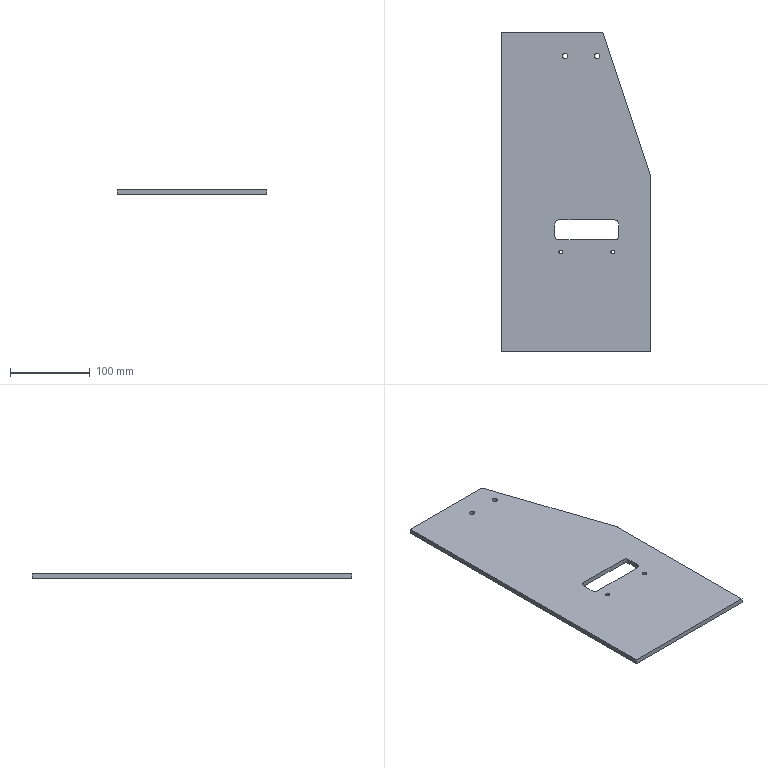Component | SolidWorks | JHK-B1003RightRearBaffle-1 | 1 solid | 25 faces | box 187 x 400 x 6 mm | volume 403848 mm3 | cylinder 14 | plane 11 | commonest cylinder face diameters 5 x4 6.8 x4 10 x4 8 x2 | material Q235A
build123d program:
from build123d import *

# Parameters (mm, degrees)
BOSS_EXTRUDE1_DEPTH = 3
M8_TAPPED_HOLE1_D   = 6.8
FILLET1_R           = 4
CUT_EXTRUDE3_DEPTH  = 221.858
M6_TAPPED_HOLE1_D   = 5


with BuildPart() as part:
    # Sketch1 → Boss-Extrude1 (new, symmetric)
    with BuildSketch(Plane.XY):
        Polygon((93.5, 200), (-33.5, 200), (-93.5, 20), (-93.5, -200), (93.5, -200), align=None)
    extrude(amount=BOSS_EXTRUDE1_DEPTH, both=True)

    # M8 Tapped Hole1 (through all)
    with Locations(Plane.XY.offset(3)):
        with Locations((13.5, 170), (-26.5, 170)):
            Hole(M8_TAPPED_HOLE1_D / 2)

    # Fillet1
    fillet1_edges = [part.edges().sort_by_distance(p)[0] for p in [
        (-93.5, 20, 0),
        (-33.5, 200, 0),
    ]]
    fillet(fillet1_edges, radius=FILLET1_R)

    # Sketch6 → Cut-Extrude3 (cut, through all)
    with BuildSketch(Plane.XY.offset(3)):
        with BuildLine():
            Line((-48.5, -60), (21.5, -60))
            ThreePointArc((21.5, -60), (25.036, -58.536), (26.5, -55))
            Line((26.5, -55), (26.5, -40))
            ThreePointArc((26.5, -40), (25.036, -36.464), (21.5, -35))
            Line((21.5, -35), (-48.5, -35))
            ThreePointArc((-48.5, -35), (-52.036, -36.464), (-53.5, -40))
            Line((-53.5, -40), (-53.5, -55))
            ThreePointArc((-53.5, -55), (-52.036, -58.536), (-48.5, -60))
        make_face()
    extrude(amount=-CUT_EXTRUDE3_DEPTH, mode=Mode.SUBTRACT)

    # M6 Tapped Hole1 (through all)
    with Locations(Plane.XY.offset(3)):
        with Locations((-46, -75), (19, -75)):
            Hole(M6_TAPPED_HOLE1_D / 2)


solid = part.part

# Placed as in the assembly
solid = solid.moved(Location((226.5, 0, -142), (-180, 0, 180)))
STEP:
#1=COLOUR_RGB('',0.7922,0.8196,0.9333);
#2=FILL_AREA_STYLE_COLOUR('',#1);
#3=FILL_AREA_STYLE('',(#2));
#4=SURFACE_STYLE_FILL_AREA(#3);
#5=SURFACE_SIDE_STYLE('',(#4));
#6=SURFACE_STYLE_USAGE(.BOTH.,#5);
#7=PRESENTATION_STYLE_ASSIGNMENT((#6));
#8=CARTESIAN_POINT('',(10.827,-2.953,-5.472));
#9=VERTEX_POINT('',#8);
#10=CARTESIAN_POINT('',(10.63,-2.953,-5.472));
#11=VERTEX_POINT('',#10);
#12=CARTESIAN_POINT('',(10.728,-2.953,-5.472));
#13=DIRECTION('',(0.,0.,-1.));
#14=DIRECTION('',(-1.,0.,0.));
#15=AXIS2_PLACEMENT_3D('',#12,#13,#14);
#16=CIRCLE('',#15,0.09843);
#17=EDGE_CURVE('',#9,#11,#16,.T.);
#18=ORIENTED_EDGE('',*,*,#17,.F.);
#19=CARTESIAN_POINT('',(10.827,-2.953,-5.709));
#20=VERTEX_POINT('',#19);
#21=CARTESIAN_POINT('',(10.827,-2.953,-5.709));
#22=DIRECTION('',(0.,0.,-1.));
#23=VECTOR('',#22,39.37);
#24=LINE('',#21,#23);
#25=EDGE_CURVE('',#9,#20,#24,.T.);
#26=ORIENTED_EDGE('',*,*,#25,.T.);
#27=CARTESIAN_POINT('',(10.63,-2.953,-5.709));
#28=VERTEX_POINT('',#27);
#29=CARTESIAN_POINT('',(10.728,-2.953,-5.709));
#30=DIRECTION('',(0.,0.,-1.));
#31=DIRECTION('',(-1.,0.,0.));
#32=AXIS2_PLACEMENT_3D('',#29,#30,#31);
#33=CIRCLE('',#32,0.09843);
#34=EDGE_CURVE('',#20,#28,#33,.T.);
#35=ORIENTED_EDGE('',*,*,#34,.T.);
#36=CARTESIAN_POINT('',(10.63,-2.953,-5.709));
#37=DIRECTION('',(0.,0.,-1.));
#38=VECTOR('',#37,39.37);
#39=LINE('',#36,#38);
#40=EDGE_CURVE('',#11,#28,#39,.T.);
#41=ORIENTED_EDGE('',*,*,#40,.F.);
#42=EDGE_LOOP('',(#18,#26,#35,#41));
#43=FACE_OUTER_BOUND('',#42,.T.);
#44=CARTESIAN_POINT('',(10.728,-2.953,-5.709));
#45=DIRECTION('',(0.,0.,-1.));
#46=DIRECTION('',(-1.,0.,0.));
#47=AXIS2_PLACEMENT_3D('',#44,#45,#46);
#48=CYLINDRICAL_SURFACE('',#47,0.09843);
#49=ADVANCED_FACE('',(#43),#48,.F.);
#50=CARTESIAN_POINT('',(8.268,-2.953,-5.472));
#51=VERTEX_POINT('',#50);
#52=CARTESIAN_POINT('',(8.071,-2.953,-5.472));
#53=VERTEX_POINT('',#52);
#54=CARTESIAN_POINT('',(8.169,-2.953,-5.472));
#55=DIRECTION('',(0.,0.,-1.));
#56=DIRECTION('',(-1.,0.,0.));
#57=AXIS2_PLACEMENT_3D('',#54,#55,#56);
#58=CIRCLE('',#57,0.09843);
#59=EDGE_CURVE('',#51,#53,#58,.T.);
#60=ORIENTED_EDGE('',*,*,#59,.F.);
#61=CARTESIAN_POINT('',(8.268,-2.953,-5.709));
#62=VERTEX_POINT('',#61);
#63=CARTESIAN_POINT('',(8.268,-2.953,-5.709));
#64=DIRECTION('',(0.,0.,-1.));
#65=VECTOR('',#64,39.37);
#66=LINE('',#63,#65);
#67=EDGE_CURVE('',#51,#62,#66,.T.);
#68=ORIENTED_EDGE('',*,*,#67,.T.);
#69=CARTESIAN_POINT('',(8.071,-2.953,-5.709));
#70=VERTEX_POINT('',#69);
#71=CARTESIAN_POINT('',(8.169,-2.953,-5.709));
#72=DIRECTION('',(0.,0.,-1.));
#73=DIRECTION('',(-1.,0.,0.));
#74=AXIS2_PLACEMENT_3D('',#71,#72,#73);
#75=CIRCLE('',#74,0.09843);
#76=EDGE_CURVE('',#62,#70,#75,.T.);
#77=ORIENTED_EDGE('',*,*,#76,.T.);
#78=CARTESIAN_POINT('',(8.071,-2.953,-5.709));
#79=DIRECTION('',(0.,0.,-1.));
#80=VECTOR('',#79,39.37);
#81=LINE('',#78,#80);
#82=EDGE_CURVE('',#53,#70,#81,.T.);
#83=ORIENTED_EDGE('',*,*,#82,.F.);
#84=EDGE_LOOP('',(#60,#68,#77,#83));
#85=FACE_OUTER_BOUND('',#84,.T.);
#86=CARTESIAN_POINT('',(8.169,-2.953,-5.709));
#87=DIRECTION('',(0.,0.,-1.));
#88=DIRECTION('',(-1.,0.,0.));
#89=AXIS2_PLACEMENT_3D('',#86,#87,#88);
#90=CYLINDRICAL_SURFACE('',#89,0.09843);
#91=ADVANCED_FACE('',(#85),#90,.F.);
#92=CARTESIAN_POINT('',(8.52,6.693,-5.472));
#93=VERTEX_POINT('',#92);
#94=CARTESIAN_POINT('',(8.252,6.693,-5.472));
#95=VERTEX_POINT('',#94);
#96=CARTESIAN_POINT('',(8.386,6.693,-5.472));
#97=DIRECTION('',(0.,0.,-1.));
#98=DIRECTION('',(-1.,0.,0.));
#99=AXIS2_PLACEMENT_3D('',#96,#97,#98);
#100=CIRCLE('',#99,0.1339);
#101=EDGE_CURVE('',#93,#95,#100,.T.);
#102=ORIENTED_EDGE('',*,*,#101,.F.);
#103=CARTESIAN_POINT('',(8.52,6.693,-5.709));
#104=VERTEX_POINT('',#103);
#105=CARTESIAN_POINT('',(8.52,6.693,-5.709));
#106=DIRECTION('',(0.,0.,-1.));
#107=VECTOR('',#106,39.37);
#108=LINE('',#105,#107);
#109=EDGE_CURVE('',#93,#104,#108,.T.);
#110=ORIENTED_EDGE('',*,*,#109,.T.);
#111=CARTESIAN_POINT('',(8.252,6.693,-5.709));
#112=VERTEX_POINT('',#111);
#113=CARTESIAN_POINT('',(8.386,6.693,-5.709));
#114=DIRECTION('',(0.,0.,-1.));
#115=DIRECTION('',(-1.,0.,0.));
#116=AXIS2_PLACEMENT_3D('',#113,#114,#115);
#117=CIRCLE('',#116,0.1339);
#118=EDGE_CURVE('',#104,#112,#117,.T.);
#119=ORIENTED_EDGE('',*,*,#118,.T.);
#120=CARTESIAN_POINT('',(8.252,6.693,-5.709));
#121=DIRECTION('',(0.,0.,-1.));
#122=VECTOR('',#121,39.37);
#123=LINE('',#120,#122);
#124=EDGE_CURVE('',#95,#112,#123,.T.);
#125=ORIENTED_EDGE('',*,*,#124,.F.);
#126=EDGE_LOOP('',(#102,#110,#119,#125));
#127=FACE_OUTER_BOUND('',#126,.T.);
#128=CARTESIAN_POINT('',(8.386,6.693,-5.709));
#129=DIRECTION('',(0.,0.,-1.));
#130=DIRECTION('',(-1.,0.,0.));
#131=AXIS2_PLACEMENT_3D('',#128,#129,#130);
#132=CYLINDRICAL_SURFACE('',#131,0.1339);
#133=ADVANCED_FACE('',(#127),#132,.F.);
#134=CARTESIAN_POINT('',(10.094,6.693,-5.472));
#135=VERTEX_POINT('',#134);
#136=CARTESIAN_POINT('',(9.827,6.693,-5.472));
#137=VERTEX_POINT('',#136);
#138=CARTESIAN_POINT('',(9.961,6.693,-5.472));
#139=DIRECTION('',(0.,0.,-1.));
#140=DIRECTION('',(-1.,0.,0.));
#141=AXIS2_PLACEMENT_3D('',#138,#139,#140);
#142=CIRCLE('',#141,0.1339);
#143=EDGE_CURVE('',#135,#137,#142,.T.);
#144=ORIENTED_EDGE('',*,*,#143,.F.);
#145=CARTESIAN_POINT('',(10.094,6.693,-5.709));
#146=VERTEX_POINT('',#145);
#147=CARTESIAN_POINT('',(10.094,6.693,-5.709));
#148=DIRECTION('',(0.,0.,-1.));
#149=VECTOR('',#148,39.37);
#150=LINE('',#147,#149);
#151=EDGE_CURVE('',#135,#146,#150,.T.);
#152=ORIENTED_EDGE('',*,*,#151,.T.);
#153=CARTESIAN_POINT('',(9.827,6.693,-5.709));
#154=VERTEX_POINT('',#153);
#155=CARTESIAN_POINT('',(9.961,6.693,-5.709));
#156=DIRECTION('',(0.,0.,-1.));
#157=DIRECTION('',(-1.,0.,0.));
#158=AXIS2_PLACEMENT_3D('',#155,#156,#157);
#159=CIRCLE('',#158,0.1339);
#160=EDGE_CURVE('',#146,#154,#159,.T.);
#161=ORIENTED_EDGE('',*,*,#160,.T.);
#162=CARTESIAN_POINT('',(9.827,6.693,-5.709));
#163=DIRECTION('',(0.,0.,-1.));
#164=VECTOR('',#163,39.37);
#165=LINE('',#162,#164);
#166=EDGE_CURVE('',#137,#154,#165,.T.);
#167=ORIENTED_EDGE('',*,*,#166,.F.);
#168=EDGE_LOOP('',(#144,#152,#161,#167));
#169=FACE_OUTER_BOUND('',#168,.T.);
#170=CARTESIAN_POINT('',(9.961,6.693,-5.709));
#171=DIRECTION('',(0.,0.,-1.));
#172=DIRECTION('',(-1.,0.,0.));
#173=AXIS2_PLACEMENT_3D('',#170,#171,#172);
#174=CYLINDRICAL_SURFACE('',#173,0.1339);
#175=ADVANCED_FACE('',(#169),#174,.F.);
#176=CARTESIAN_POINT('',(12.598,0.7618,-5.709));
#177=VERTEX_POINT('',#176);
#178=CARTESIAN_POINT('',(12.598,-7.874,-5.709));
#179=VERTEX_POINT('',#178);
#180=CARTESIAN_POINT('',(12.598,-7.874,-5.709));
#181=DIRECTION('',(0.,-1.,0.));
#182=VECTOR('',#181,39.37);
#183=LINE('',#180,#182);
#184=EDGE_CURVE('',#177,#179,#183,.T.);
#185=ORIENTED_EDGE('',*,*,#184,.F.);
#186=CARTESIAN_POINT('',(12.598,0.7618,-5.472));
#187=VERTEX_POINT('',#186);
#188=CARTESIAN_POINT('',(12.598,0.7618,-5.709));
#189=DIRECTION('',(-0.,-0.,1.));
#190=VECTOR('',#189,39.37);
#191=LINE('',#188,#190);
#192=EDGE_CURVE('',#177,#187,#191,.T.);
#193=ORIENTED_EDGE('',*,*,#192,.T.);
#194=CARTESIAN_POINT('',(12.598,-7.874,-5.472));
#195=VERTEX_POINT('',#194);
#196=CARTESIAN_POINT('',(12.598,-7.874,-5.472));
#197=DIRECTION('',(0.,-1.,0.));
#198=VECTOR('',#197,39.37);
#199=LINE('',#196,#198);
#200=EDGE_CURVE('',#187,#195,#199,.T.);
#201=ORIENTED_EDGE('',*,*,#200,.T.);
#202=CARTESIAN_POINT('',(12.598,-7.874,-5.709));
#203=DIRECTION('',(-0.,-0.,1.));
#204=VECTOR('',#203,39.37);
#205=LINE('',#202,#204);
#206=EDGE_CURVE('',#179,#195,#205,.T.);
#207=ORIENTED_EDGE('',*,*,#206,.F.);
#208=EDGE_LOOP('',(#185,#193,#201,#207));
#209=FACE_OUTER_BOUND('',#208,.T.);
#210=CARTESIAN_POINT('',(12.598,-7.874,-5.709));
#211=DIRECTION('',(-1.,-0.,-0.));
#212=DIRECTION('',(-0.,-0.,1.));
#213=AXIS2_PLACEMENT_3D('',#210,#211,#212);
#214=PLANE('',#213);
#215=ADVANCED_FACE('',(#209),#214,.F.);
#216=CARTESIAN_POINT('',(5.236,-7.874,-5.472));
#217=VERTEX_POINT('',#216);
#218=CARTESIAN_POINT('',(12.598,-7.874,-5.472));
#219=DIRECTION('',(-1.,-0.,0.));
#220=VECTOR('',#219,39.37);
#221=LINE('',#218,#220);
#222=EDGE_CURVE('',#195,#217,#221,.T.);
#223=ORIENTED_EDGE('',*,*,#222,.T.);
#224=CARTESIAN_POINT('',(5.236,-7.874,-5.709));
#225=VERTEX_POINT('',#224);
#226=CARTESIAN_POINT('',(5.236,-7.874,-5.709));
#227=DIRECTION('',(-0.,-0.,1.));
#228=VECTOR('',#227,39.37);
#229=LINE('',#226,#228);
#230=EDGE_CURVE('',#225,#217,#229,.T.);
#231=ORIENTED_EDGE('',*,*,#230,.F.);
#232=CARTESIAN_POINT('',(12.598,-7.874,-5.709));
#233=DIRECTION('',(-1.,-0.,0.));
#234=VECTOR('',#233,39.37);
#235=LINE('',#232,#234);
#236=EDGE_CURVE('',#179,#225,#235,.T.);
#237=ORIENTED_EDGE('',*,*,#236,.F.);
#238=ORIENTED_EDGE('',*,*,#206,.T.);
#239=EDGE_LOOP('',(#223,#231,#237,#238));
#240=FACE_OUTER_BOUND('',#239,.T.);
#241=CARTESIAN_POINT('',(12.598,-7.874,-5.709));
#242=DIRECTION('',(-0.,1.,0.));
#243=DIRECTION('',(0.,0.,-1.));
#244=AXIS2_PLACEMENT_3D('',#241,#242,#243);
#245=PLANE('',#244);
#246=ADVANCED_FACE('',(#240),#245,.F.);
#247=CARTESIAN_POINT('',(5.236,7.874,-5.472));
#248=VERTEX_POINT('',#247);
#249=CARTESIAN_POINT('',(5.236,7.874,-5.472));
#250=DIRECTION('',(-0.,1.,-0.));
#251=VECTOR('',#250,39.37);
#252=LINE('',#249,#251);
#253=EDGE_CURVE('',#217,#248,#252,.T.);
#254=ORIENTED_EDGE('',*,*,#253,.T.);
#255=CARTESIAN_POINT('',(5.236,7.874,-5.709));
#256=VERTEX_POINT('',#255);
#257=CARTESIAN_POINT('',(5.236,7.874,-5.709));
#258=DIRECTION('',(-0.,-0.,1.));
#259=VECTOR('',#258,39.37);
#260=LINE('',#257,#259);
#261=EDGE_CURVE('',#256,#248,#260,.T.);
#262=ORIENTED_EDGE('',*,*,#261,.F.);
#263=CARTESIAN_POINT('',(5.236,7.874,-5.709));
#264=DIRECTION('',(-0.,1.,-0.));
#265=VECTOR('',#264,39.37);
#266=LINE('',#263,#265);
#267=EDGE_CURVE('',#225,#256,#266,.T.);
#268=ORIENTED_EDGE('',*,*,#267,.F.);
#269=ORIENTED_EDGE('',*,*,#230,.T.);
#270=EDGE_LOOP('',(#254,#262,#268,#269));
#271=FACE_OUTER_BOUND('',#270,.T.);
#272=CARTESIAN_POINT('',(5.236,7.874,-5.709));
#273=DIRECTION('',(1.,0.,0.));
#274=DIRECTION('',(0.,0.,-1.));
#275=AXIS2_PLACEMENT_3D('',#272,#273,#274);
#276=PLANE('',#275);
#277=ADVANCED_FACE('',(#271),#276,.F.);
#278=CARTESIAN_POINT('',(10.123,7.874,-5.472));
#279=VERTEX_POINT('',#278);
#280=CARTESIAN_POINT('',(5.236,7.874,-5.472));
#281=DIRECTION('',(1.,0.,-0.));
#282=VECTOR('',#281,39.37);
#283=LINE('',#280,#282);
#284=EDGE_CURVE('',#248,#279,#283,.T.);
#285=ORIENTED_EDGE('',*,*,#284,.T.);
#286=CARTESIAN_POINT('',(10.123,7.874,-5.709));
#287=VERTEX_POINT('',#286);
#288=CARTESIAN_POINT('',(10.123,7.874,-5.709));
#289=DIRECTION('',(0.,0.,-1.));
#290=VECTOR('',#289,39.37);
#291=LINE('',#288,#290);
#292=EDGE_CURVE('',#279,#287,#291,.T.);
#293=ORIENTED_EDGE('',*,*,#292,.T.);
#294=CARTESIAN_POINT('',(5.236,7.874,-5.709));
#295=DIRECTION('',(1.,0.,-0.));
#296=VECTOR('',#295,39.37);
#297=LINE('',#294,#296);
#298=EDGE_CURVE('',#256,#287,#297,.T.);
#299=ORIENTED_EDGE('',*,*,#298,.F.);
#300=ORIENTED_EDGE('',*,*,#261,.T.);
#301=EDGE_LOOP('',(#285,#293,#299,#300));
#302=FACE_OUTER_BOUND('',#301,.T.);
#303=CARTESIAN_POINT('',(5.236,7.874,-5.709));
#304=DIRECTION('',(0.,-1.,0.));
#305=DIRECTION('',(-1.,-0.,0.));
#306=AXIS2_PLACEMENT_3D('',#303,#304,#305);
#307=PLANE('',#306);
#308=ADVANCED_FACE('',(#302),#307,.F.);
#309=CARTESIAN_POINT('',(10.272,7.766,-5.472));
#310=VERTEX_POINT('',#309);
#311=CARTESIAN_POINT('',(12.59,0.8116,-5.472));
#312=VERTEX_POINT('',#311);
#313=CARTESIAN_POINT('',(12.598,0.7874,-5.472));
#314=DIRECTION('',(0.3162,-0.9487,0.));
#315=VECTOR('',#314,39.37);
#316=LINE('',#313,#315);
#317=EDGE_CURVE('',#310,#312,#316,.T.);
#318=ORIENTED_EDGE('',*,*,#317,.T.);
#319=CARTESIAN_POINT('',(12.59,0.8116,-5.709));
#320=VERTEX_POINT('',#319);
#321=CARTESIAN_POINT('',(12.59,0.8116,-5.709));
#322=DIRECTION('',(0.,0.,-1.));
#323=VECTOR('',#322,39.37);
#324=LINE('',#321,#323);
#325=EDGE_CURVE('',#312,#320,#324,.T.);
#326=ORIENTED_EDGE('',*,*,#325,.T.);
#327=CARTESIAN_POINT('',(10.272,7.766,-5.709));
#328=VERTEX_POINT('',#327);
#329=CARTESIAN_POINT('',(12.598,0.7874,-5.709));
#330=DIRECTION('',(0.3162,-0.9487,0.));
#331=VECTOR('',#330,39.37);
#332=LINE('',#329,#331);
#333=EDGE_CURVE('',#328,#320,#332,.T.);
#334=ORIENTED_EDGE('',*,*,#333,.F.);
#335=CARTESIAN_POINT('',(10.272,7.766,-5.709));
#336=DIRECTION('',(-0.,-0.,1.));
#337=VECTOR('',#336,39.37);
#338=LINE('',#335,#337);
#339=EDGE_CURVE('',#328,#310,#338,.T.);
#340=ORIENTED_EDGE('',*,*,#339,.T.);
#341=EDGE_LOOP('',(#318,#326,#334,#340));
#342=FACE_OUTER_BOUND('',#341,.T.);
#343=CARTESIAN_POINT('',(12.598,0.7874,-5.709));
#344=DIRECTION('',(-0.9487,-0.3162,0.));
#345=DIRECTION('',(-0.3162,0.9487,-0.));
#346=AXIS2_PLACEMENT_3D('',#343,#344,#345);
#347=PLANE('',#346);
#348=ADVANCED_FACE('',(#342),#347,.F.);
#349=CARTESIAN_POINT('',(10.728,-2.953,-5.709));
#350=DIRECTION('',(0.,0.,-1.));
#351=DIRECTION('',(-1.,0.,0.));
#352=AXIS2_PLACEMENT_3D('',#349,#350,#351);
#353=CIRCLE('',#352,0.09843);
#354=EDGE_CURVE('',#28,#20,#353,.T.);
#355=ORIENTED_EDGE('',*,*,#354,.F.);
#356=ORIENTED_EDGE('',*,*,#34,.F.);
#357=EDGE_LOOP('',(#355,#356));
#358=FACE_BOUND('',#357,.T.);
#359=CARTESIAN_POINT('',(8.169,-2.953,-5.709));
#360=DIRECTION('',(0.,0.,-1.));
#361=DIRECTION('',(-1.,0.,0.));
#362=AXIS2_PLACEMENT_3D('',#359,#360,#361);
#363=CIRCLE('',#362,0.09843);
#364=EDGE_CURVE('',#70,#62,#363,.T.);
#365=ORIENTED_EDGE('',*,*,#364,.F.);
#366=ORIENTED_EDGE('',*,*,#76,.F.);
#367=EDGE_LOOP('',(#365,#366));
#368=FACE_BOUND('',#367,.T.);
#369=CARTESIAN_POINT('',(7.874,-1.575,-5.709));
#370=VERTEX_POINT('',#369);
#371=CARTESIAN_POINT('',(8.071,-1.378,-5.709));
#372=VERTEX_POINT('',#371);
#373=CARTESIAN_POINT('',(8.071,-1.575,-5.709));
#374=DIRECTION('',(0.,0.,-1.));
#375=DIRECTION('',(-1.,0.,0.));
#376=AXIS2_PLACEMENT_3D('',#373,#374,#375);
#377=CIRCLE('',#376,0.1969);
#378=EDGE_CURVE('',#370,#372,#377,.T.);
#379=ORIENTED_EDGE('',*,*,#378,.F.);
#380=CARTESIAN_POINT('',(7.874,-2.165,-5.709));
#381=VERTEX_POINT('',#380);
#382=CARTESIAN_POINT('',(7.874,-2.165,-5.709));
#383=DIRECTION('',(-0.,1.,-0.));
#384=VECTOR('',#383,39.37);
#385=LINE('',#382,#384);
#386=EDGE_CURVE('',#381,#370,#385,.T.);
#387=ORIENTED_EDGE('',*,*,#386,.F.);
#388=CARTESIAN_POINT('',(8.071,-2.362,-5.709));
#389=VERTEX_POINT('',#388);
#390=CARTESIAN_POINT('',(8.071,-2.165,-5.709));
#391=DIRECTION('',(0.,0.,-1.));
#392=DIRECTION('',(-1.,0.,0.));
#393=AXIS2_PLACEMENT_3D('',#390,#391,#392);
#394=CIRCLE('',#393,0.1969);
#395=EDGE_CURVE('',#389,#381,#394,.T.);
#396=ORIENTED_EDGE('',*,*,#395,.F.);
#397=CARTESIAN_POINT('',(10.827,-2.362,-5.709));
#398=VERTEX_POINT('',#397);
#399=CARTESIAN_POINT('',(10.827,-2.362,-5.709));
#400=DIRECTION('',(-1.,-0.,0.));
#401=VECTOR('',#400,39.37);
#402=LINE('',#399,#401);
#403=EDGE_CURVE('',#398,#389,#402,.T.);
#404=ORIENTED_EDGE('',*,*,#403,.F.);
#405=CARTESIAN_POINT('',(11.024,-2.165,-5.709));
#406=VERTEX_POINT('',#405);
#407=CARTESIAN_POINT('',(10.827,-2.165,-5.709));
#408=DIRECTION('',(0.,0.,-1.));
#409=DIRECTION('',(-1.,0.,0.));
#410=AXIS2_PLACEMENT_3D('',#407,#408,#409);
#411=CIRCLE('',#410,0.1969);
#412=EDGE_CURVE('',#406,#398,#411,.T.);
#413=ORIENTED_EDGE('',*,*,#412,.F.);
#414=CARTESIAN_POINT('',(11.024,-1.575,-5.709));
#415=VERTEX_POINT('',#414);
#416=CARTESIAN_POINT('',(11.024,-2.165,-5.709));
#417=DIRECTION('',(0.,-1.,0.));
#418=VECTOR('',#417,39.37);
#419=LINE('',#416,#418);
#420=EDGE_CURVE('',#415,#406,#419,.T.);
#421=ORIENTED_EDGE('',*,*,#420,.F.);
#422=CARTESIAN_POINT('',(10.827,-1.378,-5.709));
#423=VERTEX_POINT('',#422);
#424=CARTESIAN_POINT('',(10.827,-1.575,-5.709));
#425=DIRECTION('',(0.,0.,-1.));
#426=DIRECTION('',(1.,0.,0.));
#427=AXIS2_PLACEMENT_3D('',#424,#425,#426);
#428=CIRCLE('',#427,0.1969);
#429=EDGE_CURVE('',#423,#415,#428,.T.);
#430=ORIENTED_EDGE('',*,*,#429,.F.);
#431=CARTESIAN_POINT('',(10.827,-1.378,-5.709));
#432=DIRECTION('',(1.,0.,-0.));
#433=VECTOR('',#432,39.37);
#434=LINE('',#431,#433);
#435=EDGE_CURVE('',#372,#423,#434,.T.);
#436=ORIENTED_EDGE('',*,*,#435,.F.);
#437=EDGE_LOOP('',(#379,#387,#396,#404,#413,#421,#430,#436));
#438=FACE_BOUND('',#437,.T.);
#439=CARTESIAN_POINT('',(8.386,6.693,-5.709));
#440=DIRECTION('',(0.,0.,-1.));
#441=DIRECTION('',(-1.,0.,0.));
#442=AXIS2_PLACEMENT_3D('',#439,#440,#441);
#443=CIRCLE('',#442,0.1339);
#444=EDGE_CURVE('',#112,#104,#443,.T.);
#445=ORIENTED_EDGE('',*,*,#444,.F.);
#446=ORIENTED_EDGE('',*,*,#118,.F.);
#447=EDGE_LOOP('',(#445,#446));
#448=FACE_BOUND('',#447,.T.);
#449=CARTESIAN_POINT('',(9.961,6.693,-5.709));
#450=DIRECTION('',(0.,0.,-1.));
#451=DIRECTION('',(-1.,0.,0.));
#452=AXIS2_PLACEMENT_3D('',#449,#450,#451);
#453=CIRCLE('',#452,0.1339);
#454=EDGE_CURVE('',#154,#146,#453,.T.);
#455=ORIENTED_EDGE('',*,*,#454,.F.);
#456=ORIENTED_EDGE('',*,*,#160,.F.);
#457=EDGE_LOOP('',(#455,#456));
#458=FACE_BOUND('',#457,.T.);
#459=ORIENTED_EDGE('',*,*,#333,.T.);
#460=CARTESIAN_POINT('',(12.441,0.7618,-5.709));
#461=DIRECTION('',(0.,0.,-1.));
#462=DIRECTION('',(-1.,0.,0.));
#463=AXIS2_PLACEMENT_3D('',#460,#461,#462);
#464=CIRCLE('',#463,0.1575);
#465=EDGE_CURVE('',#320,#177,#464,.T.);
#466=ORIENTED_EDGE('',*,*,#465,.T.);
#467=ORIENTED_EDGE('',*,*,#184,.T.);
#468=ORIENTED_EDGE('',*,*,#236,.T.);
#469=ORIENTED_EDGE('',*,*,#267,.T.);
#470=ORIENTED_EDGE('',*,*,#298,.T.);
#471=CARTESIAN_POINT('',(10.123,7.717,-5.709));
#472=DIRECTION('',(0.,0.,-1.));
#473=DIRECTION('',(-1.,0.,0.));
#474=AXIS2_PLACEMENT_3D('',#471,#472,#473);
#475=CIRCLE('',#474,0.1575);
#476=EDGE_CURVE('',#287,#328,#475,.T.);
#477=ORIENTED_EDGE('',*,*,#476,.T.);
#478=EDGE_LOOP('',(#459,#466,#467,#468,#469,#470,#477));
#479=FACE_OUTER_BOUND('',#478,.T.);
#480=CARTESIAN_POINT('',(8.917,0.,-5.709));
#481=DIRECTION('',(-0.,0.,-1.));
#482=DIRECTION('',(-1.,-0.,0.));
#483=AXIS2_PLACEMENT_3D('',#480,#481,#482);
#484=PLANE('',#483);
#485=ADVANCED_FACE('',(#358,#368,#438,#448,#458,#479),#484,.T.);
#486=CARTESIAN_POINT('',(10.728,-2.953,-5.472));
#487=DIRECTION('',(0.,0.,-1.));
#488=DIRECTION('',(-1.,0.,0.));
#489=AXIS2_PLACEMENT_3D('',#486,#487,#488);
#490=CIRCLE('',#489,0.09843);
#491=EDGE_CURVE('',#11,#9,#490,.T.);
#492=ORIENTED_EDGE('',*,*,#491,.T.);
#493=ORIENTED_EDGE('',*,*,#17,.T.);
#494=EDGE_LOOP('',(#492,#493));
#495=FACE_BOUND('',#494,.T.);
#496=CARTESIAN_POINT('',(8.169,-2.953,-5.472));
#497=DIRECTION('',(0.,0.,-1.));
#498=DIRECTION('',(-1.,0.,0.));
#499=AXIS2_PLACEMENT_3D('',#496,#497,#498);
#500=CIRCLE('',#499,0.09843);
#501=EDGE_CURVE('',#53,#51,#500,.T.);
#502=ORIENTED_EDGE('',*,*,#501,.T.);
#503=ORIENTED_EDGE('',*,*,#59,.T.);
#504=EDGE_LOOP('',(#502,#503));
#505=FACE_BOUND('',#504,.T.);
#506=CARTESIAN_POINT('',(7.874,-2.165,-5.472));
#507=VERTEX_POINT('',#506);
#508=CARTESIAN_POINT('',(7.874,-1.575,-5.472));
#509=VERTEX_POINT('',#508);
#510=CARTESIAN_POINT('',(7.874,-2.165,-5.472));
#511=DIRECTION('',(-0.,1.,-0.));
#512=VECTOR('',#511,39.37);
#513=LINE('',#510,#512);
#514=EDGE_CURVE('',#507,#509,#513,.T.);
#515=ORIENTED_EDGE('',*,*,#514,.T.);
#516=CARTESIAN_POINT('',(8.071,-1.378,-5.472));
#517=VERTEX_POINT('',#516);
#518=CARTESIAN_POINT('',(8.071,-1.575,-5.472));
#519=DIRECTION('',(0.,0.,-1.));
#520=DIRECTION('',(-1.,0.,0.));
#521=AXIS2_PLACEMENT_3D('',#518,#519,#520);
#522=CIRCLE('',#521,0.1969);
#523=EDGE_CURVE('',#509,#517,#522,.T.);
#524=ORIENTED_EDGE('',*,*,#523,.T.);
#525=CARTESIAN_POINT('',(10.827,-1.378,-5.472));
#526=VERTEX_POINT('',#525);
#527=CARTESIAN_POINT('',(10.827,-1.378,-5.472));
#528=DIRECTION('',(1.,0.,-0.));
#529=VECTOR('',#528,39.37);
#530=LINE('',#527,#529);
#531=EDGE_CURVE('',#517,#526,#530,.T.);
#532=ORIENTED_EDGE('',*,*,#531,.T.);
#533=CARTESIAN_POINT('',(11.024,-1.575,-5.472));
#534=VERTEX_POINT('',#533);
#535=CARTESIAN_POINT('',(10.827,-1.575,-5.472));
#536=DIRECTION('',(0.,0.,-1.));
#537=DIRECTION('',(1.,0.,0.));
#538=AXIS2_PLACEMENT_3D('',#535,#536,#537);
#539=CIRCLE('',#538,0.1969);
#540=EDGE_CURVE('',#526,#534,#539,.T.);
#541=ORIENTED_EDGE('',*,*,#540,.T.);
#542=CARTESIAN_POINT('',(11.024,-2.165,-5.472));
#543=VERTEX_POINT('',#542);
#544=CARTESIAN_POINT('',(11.024,-2.165,-5.472));
#545=DIRECTION('',(0.,-1.,0.));
#546=VECTOR('',#545,39.37);
#547=LINE('',#544,#546);
#548=EDGE_CURVE('',#534,#543,#547,.T.);
#549=ORIENTED_EDGE('',*,*,#548,.T.);
#550=CARTESIAN_POINT('',(10.827,-2.362,-5.472));
#551=VERTEX_POINT('',#550);
#552=CARTESIAN_POINT('',(10.827,-2.165,-5.472));
#553=DIRECTION('',(0.,0.,-1.));
#554=DIRECTION('',(-1.,0.,0.));
#555=AXIS2_PLACEMENT_3D('',#552,#553,#554);
#556=CIRCLE('',#555,0.1969);
#557=EDGE_CURVE('',#543,#551,#556,.T.);
#558=ORIENTED_EDGE('',*,*,#557,.T.);
#559=CARTESIAN_POINT('',(8.071,-2.362,-5.472));
#560=VERTEX_POINT('',#559);
#561=CARTESIAN_POINT('',(10.827,-2.362,-5.472));
#562=DIRECTION('',(-1.,-0.,0.));
#563=VECTOR('',#562,39.37);
#564=LINE('',#561,#563);
#565=EDGE_CURVE('',#551,#560,#564,.T.);
#566=ORIENTED_EDGE('',*,*,#565,.T.);
#567=CARTESIAN_POINT('',(8.071,-2.165,-5.472));
#568=DIRECTION('',(0.,0.,-1.));
#569=DIRECTION('',(-1.,0.,0.));
#570=AXIS2_PLACEMENT_3D('',#567,#568,#569);
#571=CIRCLE('',#570,0.1969);
#572=EDGE_CURVE('',#560,#507,#571,.T.);
#573=ORIENTED_EDGE('',*,*,#572,.T.);
#574=EDGE_LOOP('',(#515,#524,#532,#541,#549,#558,#566,#573));
#575=FACE_BOUND('',#574,.T.);
#576=CARTESIAN_POINT('',(8.386,6.693,-5.472));
#577=DIRECTION('',(0.,0.,-1.));
#578=DIRECTION('',(-1.,0.,0.));
#579=AXIS2_PLACEMENT_3D('',#576,#577,#578);
#580=CIRCLE('',#579,0.1339);
#581=EDGE_CURVE('',#95,#93,#580,.T.);
#582=ORIENTED_EDGE('',*,*,#581,.T.);
#583=ORIENTED_EDGE('',*,*,#101,.T.);
#584=EDGE_LOOP('',(#582,#583));
#585=FACE_BOUND('',#584,.T.);
#586=CARTESIAN_POINT('',(9.961,6.693,-5.472));
#587=DIRECTION('',(0.,0.,-1.));
#588=DIRECTION('',(-1.,0.,0.));
#589=AXIS2_PLACEMENT_3D('',#586,#587,#588);
#590=CIRCLE('',#589,0.1339);
#591=EDGE_CURVE('',#137,#135,#590,.T.);
#592=ORIENTED_EDGE('',*,*,#591,.T.);
#593=ORIENTED_EDGE('',*,*,#143,.T.);
#594=EDGE_LOOP('',(#592,#593));
#595=FACE_BOUND('',#594,.T.);
#596=ORIENTED_EDGE('',*,*,#200,.F.);
#597=CARTESIAN_POINT('',(12.441,0.7618,-5.472));
#598=DIRECTION('',(-0.,-0.,1.));
#599=DIRECTION('',(-1.,0.,0.));
#600=AXIS2_PLACEMENT_3D('',#597,#598,#599);
#601=CIRCLE('',#600,0.1575);
#602=EDGE_CURVE('',#187,#312,#601,.T.);
#603=ORIENTED_EDGE('',*,*,#602,.T.);
#604=ORIENTED_EDGE('',*,*,#317,.F.);
#605=CARTESIAN_POINT('',(10.123,7.717,-5.472));
#606=DIRECTION('',(-0.,-0.,1.));
#607=DIRECTION('',(-1.,0.,0.));
#608=AXIS2_PLACEMENT_3D('',#605,#606,#607);
#609=CIRCLE('',#608,0.1575);
#610=EDGE_CURVE('',#310,#279,#609,.T.);
#611=ORIENTED_EDGE('',*,*,#610,.T.);
#612=ORIENTED_EDGE('',*,*,#284,.F.);
#613=ORIENTED_EDGE('',*,*,#253,.F.);
#614=ORIENTED_EDGE('',*,*,#222,.F.);
#615=EDGE_LOOP('',(#596,#603,#604,#611,#612,#613,#614));
#616=FACE_OUTER_BOUND('',#615,.T.);
#617=CARTESIAN_POINT('',(8.917,0.,-5.472));
#618=DIRECTION('',(-0.,0.,-1.));
#619=DIRECTION('',(-1.,-0.,0.));
#620=AXIS2_PLACEMENT_3D('',#617,#618,#619);
#621=PLANE('',#620);
#622=ADVANCED_FACE('',(#495,#505,#575,#585,#595,#616),#621,.F.);
#623=ORIENTED_EDGE('',*,*,#151,.F.);
#624=ORIENTED_EDGE('',*,*,#591,.F.);
#625=ORIENTED_EDGE('',*,*,#166,.T.);
#626=ORIENTED_EDGE('',*,*,#454,.T.);
#627=EDGE_LOOP('',(#623,#624,#625,#626));
#628=FACE_OUTER_BOUND('',#627,.T.);
#629=CARTESIAN_POINT('',(9.961,6.693,-5.709));
#630=DIRECTION('',(0.,0.,-1.));
#631=DIRECTION('',(-1.,0.,0.));
#632=AXIS2_PLACEMENT_3D('',#629,#630,#631);
#633=CYLINDRICAL_SURFACE('',#632,0.1339);
#634=ADVANCED_FACE('',(#628),#633,.F.);
#635=ORIENTED_EDGE('',*,*,#109,.F.);
#636=ORIENTED_EDGE('',*,*,#581,.F.);
#637=ORIENTED_EDGE('',*,*,#124,.T.);
#638=ORIENTED_EDGE('',*,*,#444,.T.);
#639=EDGE_LOOP('',(#635,#636,#637,#638));
#640=FACE_OUTER_BOUND('',#639,.T.);
#641=CARTESIAN_POINT('',(8.386,6.693,-5.709));
#642=DIRECTION('',(0.,0.,-1.));
#643=DIRECTION('',(-1.,0.,0.));
#644=AXIS2_PLACEMENT_3D('',#641,#642,#643);
#645=CYLINDRICAL_SURFACE('',#644,0.1339);
#646=ADVANCED_FACE('',(#640),#645,.F.);
#647=ORIENTED_EDGE('',*,*,#465,.F.);
#648=ORIENTED_EDGE('',*,*,#325,.F.);
#649=ORIENTED_EDGE('',*,*,#602,.F.);
#650=ORIENTED_EDGE('',*,*,#192,.F.);
#651=EDGE_LOOP('',(#647,#648,#649,#650));
#652=FACE_OUTER_BOUND('',#651,.T.);
#653=CARTESIAN_POINT('',(12.441,0.7618,-5.709));
#654=DIRECTION('',(-0.,-0.,1.));
#655=DIRECTION('',(1.,0.,0.));
#656=AXIS2_PLACEMENT_3D('',#653,#654,#655);
#657=CYLINDRICAL_SURFACE('',#656,0.1575);
#658=ADVANCED_FACE('',(#652),#657,.T.);
#659=ORIENTED_EDGE('',*,*,#476,.F.);
#660=ORIENTED_EDGE('',*,*,#292,.F.);
#661=ORIENTED_EDGE('',*,*,#610,.F.);
#662=ORIENTED_EDGE('',*,*,#339,.F.);
#663=EDGE_LOOP('',(#659,#660,#661,#662));
#664=FACE_OUTER_BOUND('',#663,.T.);
#665=CARTESIAN_POINT('',(10.123,7.717,-5.709));
#666=DIRECTION('',(-0.,-0.,1.));
#667=DIRECTION('',(1.,0.,0.));
#668=AXIS2_PLACEMENT_3D('',#665,#666,#667);
#669=CYLINDRICAL_SURFACE('',#668,0.1575);
#670=ADVANCED_FACE('',(#664),#669,.T.);
#671=ORIENTED_EDGE('',*,*,#378,.T.);
#672=CARTESIAN_POINT('',(8.071,-1.378,-5.472));
#673=DIRECTION('',(0.,0.,-1.));
#674=VECTOR('',#673,39.37);
#675=LINE('',#672,#674);
#676=EDGE_CURVE('',#517,#372,#675,.T.);
#677=ORIENTED_EDGE('',*,*,#676,.F.);
#678=ORIENTED_EDGE('',*,*,#523,.F.);
#679=CARTESIAN_POINT('',(7.874,-1.575,-5.472));
#680=DIRECTION('',(0.,0.,-1.));
#681=VECTOR('',#680,39.37);
#682=LINE('',#679,#681);
#683=EDGE_CURVE('',#509,#370,#682,.T.);
#684=ORIENTED_EDGE('',*,*,#683,.T.);
#685=EDGE_LOOP('',(#671,#677,#678,#684));
#686=FACE_OUTER_BOUND('',#685,.T.);
#687=CARTESIAN_POINT('',(8.071,-1.575,-5.472));
#688=DIRECTION('',(0.,0.,-1.));
#689=DIRECTION('',(-1.,0.,0.));
#690=AXIS2_PLACEMENT_3D('',#687,#688,#689);
#691=CYLINDRICAL_SURFACE('',#690,0.1969);
#692=ADVANCED_FACE('',(#686),#691,.F.);
#693=ORIENTED_EDGE('',*,*,#386,.T.);
#694=ORIENTED_EDGE('',*,*,#683,.F.);
#695=ORIENTED_EDGE('',*,*,#514,.F.);
#696=CARTESIAN_POINT('',(7.874,-2.165,-5.472));
#697=DIRECTION('',(0.,0.,-1.));
#698=VECTOR('',#697,39.37);
#699=LINE('',#696,#698);
#700=EDGE_CURVE('',#507,#381,#699,.T.);
#701=ORIENTED_EDGE('',*,*,#700,.T.);
#702=EDGE_LOOP('',(#693,#694,#695,#701));
#703=FACE_OUTER_BOUND('',#702,.T.);
#704=CARTESIAN_POINT('',(7.874,-2.165,-5.472));
#705=DIRECTION('',(-1.,-0.,-0.));
#706=DIRECTION('',(-0.,-0.,1.));
#707=AXIS2_PLACEMENT_3D('',#704,#705,#706);
#708=PLANE('',#707);
#709=ADVANCED_FACE('',(#703),#708,.F.);
#710=ORIENTED_EDGE('',*,*,#395,.T.);
#711=ORIENTED_EDGE('',*,*,#700,.F.);
#712=ORIENTED_EDGE('',*,*,#572,.F.);
#713=CARTESIAN_POINT('',(8.071,-2.362,-5.472));
#714=DIRECTION('',(0.,0.,-1.));
#715=VECTOR('',#714,39.37);
#716=LINE('',#713,#715);
#717=EDGE_CURVE('',#560,#389,#716,.T.);
#718=ORIENTED_EDGE('',*,*,#717,.T.);
#719=EDGE_LOOP('',(#710,#711,#712,#718));
#720=FACE_OUTER_BOUND('',#719,.T.);
#721=CARTESIAN_POINT('',(8.071,-2.165,-5.472));
#722=DIRECTION('',(0.,0.,-1.));
#723=DIRECTION('',(-1.,0.,0.));
#724=AXIS2_PLACEMENT_3D('',#721,#722,#723);
#725=CYLINDRICAL_SURFACE('',#724,0.1969);
#726=ADVANCED_FACE('',(#720),#725,.F.);
#727=ORIENTED_EDGE('',*,*,#403,.T.);
#728=ORIENTED_EDGE('',*,*,#717,.F.);
#729=ORIENTED_EDGE('',*,*,#565,.F.);
#730=CARTESIAN_POINT('',(10.827,-2.362,-5.472));
#731=DIRECTION('',(0.,0.,-1.));
#732=VECTOR('',#731,39.37);
#733=LINE('',#730,#732);
#734=EDGE_CURVE('',#551,#398,#733,.T.);
#735=ORIENTED_EDGE('',*,*,#734,.T.);
#736=EDGE_LOOP('',(#727,#728,#729,#735));
#737=FACE_OUTER_BOUND('',#736,.T.);
#738=CARTESIAN_POINT('',(10.827,-2.362,-5.472));
#739=DIRECTION('',(0.,-1.,-0.));
#740=DIRECTION('',(-0.,-0.,1.));
#741=AXIS2_PLACEMENT_3D('',#738,#739,#740);
#742=PLANE('',#741);
#743=ADVANCED_FACE('',(#737),#742,.F.);
#744=ORIENTED_EDGE('',*,*,#412,.T.);
#745=ORIENTED_EDGE('',*,*,#734,.F.);
#746=ORIENTED_EDGE('',*,*,#557,.F.);
#747=CARTESIAN_POINT('',(11.024,-2.165,-5.472));
#748=DIRECTION('',(0.,0.,-1.));
#749=VECTOR('',#748,39.37);
#750=LINE('',#747,#749);
#751=EDGE_CURVE('',#543,#406,#750,.T.);
#752=ORIENTED_EDGE('',*,*,#751,.T.);
#753=EDGE_LOOP('',(#744,#745,#746,#752));
#754=FACE_OUTER_BOUND('',#753,.T.);
#755=CARTESIAN_POINT('',(10.827,-2.165,-5.472));
#756=DIRECTION('',(0.,0.,-1.));
#757=DIRECTION('',(-1.,0.,0.));
#758=AXIS2_PLACEMENT_3D('',#755,#756,#757);
#759=CYLINDRICAL_SURFACE('',#758,0.1969);
#760=ADVANCED_FACE('',(#754),#759,.F.);
#761=ORIENTED_EDGE('',*,*,#420,.T.);
#762=ORIENTED_EDGE('',*,*,#751,.F.);
#763=ORIENTED_EDGE('',*,*,#548,.F.);
#764=CARTESIAN_POINT('',(11.024,-1.575,-5.472));
#765=DIRECTION('',(0.,0.,-1.));
#766=VECTOR('',#765,39.37);
#767=LINE('',#764,#766);
#768=EDGE_CURVE('',#534,#415,#767,.T.);
#769=ORIENTED_EDGE('',*,*,#768,.T.);
#770=EDGE_LOOP('',(#761,#762,#763,#769));
#771=FACE_OUTER_BOUND('',#770,.T.);
#772=CARTESIAN_POINT('',(11.024,-2.165,-5.472));
#773=DIRECTION('',(1.,0.,0.));
#774=DIRECTION('',(0.,0.,-1.));
#775=AXIS2_PLACEMENT_3D('',#772,#773,#774);
#776=PLANE('',#775);
#777=ADVANCED_FACE('',(#771),#776,.F.);
#778=ORIENTED_EDGE('',*,*,#429,.T.);
#779=ORIENTED_EDGE('',*,*,#768,.F.);
#780=ORIENTED_EDGE('',*,*,#540,.F.);
#781=CARTESIAN_POINT('',(10.827,-1.378,-5.472));
#782=DIRECTION('',(0.,0.,-1.));
#783=VECTOR('',#782,39.37);
#784=LINE('',#781,#783);
#785=EDGE_CURVE('',#526,#423,#784,.T.);
#786=ORIENTED_EDGE('',*,*,#785,.T.);
#787=EDGE_LOOP('',(#778,#779,#780,#786));
#788=FACE_OUTER_BOUND('',#787,.T.);
#789=CARTESIAN_POINT('',(10.827,-1.575,-5.472));
#790=DIRECTION('',(0.,0.,-1.));
#791=DIRECTION('',(-1.,0.,0.));
#792=AXIS2_PLACEMENT_3D('',#789,#790,#791);
#793=CYLINDRICAL_SURFACE('',#792,0.1969);
#794=ADVANCED_FACE('',(#788),#793,.F.);
#795=ORIENTED_EDGE('',*,*,#435,.T.);
#796=ORIENTED_EDGE('',*,*,#785,.F.);
#797=ORIENTED_EDGE('',*,*,#531,.F.);
#798=ORIENTED_EDGE('',*,*,#676,.T.);
#799=EDGE_LOOP('',(#795,#796,#797,#798));
#800=FACE_OUTER_BOUND('',#799,.T.);
#801=CARTESIAN_POINT('',(10.827,-1.378,-5.472));
#802=DIRECTION('',(-0.,1.,0.));
#803=DIRECTION('',(0.,0.,-1.));
#804=AXIS2_PLACEMENT_3D('',#801,#802,#803);
#805=PLANE('',#804);
#806=ADVANCED_FACE('',(#800),#805,.F.);
#807=ORIENTED_EDGE('',*,*,#67,.F.);
#808=ORIENTED_EDGE('',*,*,#501,.F.);
#809=ORIENTED_EDGE('',*,*,#82,.T.);
#810=ORIENTED_EDGE('',*,*,#364,.T.);
#811=EDGE_LOOP('',(#807,#808,#809,#810));
#812=FACE_OUTER_BOUND('',#811,.T.);
#813=CARTESIAN_POINT('',(8.169,-2.953,-5.709));
#814=DIRECTION('',(0.,0.,-1.));
#815=DIRECTION('',(-1.,0.,0.));
#816=AXIS2_PLACEMENT_3D('',#813,#814,#815);
#817=CYLINDRICAL_SURFACE('',#816,0.09843);
#818=ADVANCED_FACE('',(#812),#817,.F.);
#819=ORIENTED_EDGE('',*,*,#25,.F.);
#820=ORIENTED_EDGE('',*,*,#491,.F.);
#821=ORIENTED_EDGE('',*,*,#40,.T.);
#822=ORIENTED_EDGE('',*,*,#354,.T.);
#823=EDGE_LOOP('',(#819,#820,#821,#822));
#824=FACE_OUTER_BOUND('',#823,.T.);
#825=CARTESIAN_POINT('',(10.728,-2.953,-5.709));
#826=DIRECTION('',(0.,0.,-1.));
#827=DIRECTION('',(-1.,0.,0.));
#828=AXIS2_PLACEMENT_3D('',#825,#826,#827);
#829=CYLINDRICAL_SURFACE('',#828,0.09843);
#830=ADVANCED_FACE('',(#824),#829,.F.);
#831=CLOSED_SHELL('',(#49,#91,#133,#175,#215,#246,#277,#308,#348,#485,#622,#634,#646,#658,#670,#692,#709,#726,#743,#760,#777,#794,#806,#818,#830));
#832=MANIFOLD_SOLID_BREP('',#831);
#833=STYLED_ITEM('',(#7),#832);
#834=(LENGTH_UNIT()NAMED_UNIT(*)SI_UNIT($,.METRE.));
#835=LENGTH_MEASURE_WITH_UNIT(LENGTH_MEASURE(0.0254),#834);
#836=DIMENSIONAL_EXPONENTS(1.,0.,0.,0.,0.,0.,0.);
#837=(CONVERSION_BASED_UNIT('',#835)LENGTH_UNIT()NAMED_UNIT(#836));
#838=UNCERTAINTY_MEASURE_WITH_UNIT(LENGTH_MEASURE(0.00001),#837,'','');
#839=(NAMED_UNIT(*)PLANE_ANGLE_UNIT()SI_UNIT($,.RADIAN.));
#840=(NAMED_UNIT(*)SI_UNIT($,.STERADIAN.)SOLID_ANGLE_UNIT());
#841=(GEOMETRIC_REPRESENTATION_CONTEXT(3)GLOBAL_UNCERTAINTY_ASSIGNED_CONTEXT((#838))GLOBAL_UNIT_ASSIGNED_CONTEXT((#837,#839,#840))REPRESENTATION_CONTEXT('',''));
#842=MECHANICAL_DESIGN_GEOMETRIC_PRESENTATION_REPRESENTATION('',(#833),#841);
#843=PRESENTATION_LAYER_ASSIGNMENT('','',(#833));
#844=CARTESIAN_POINT('',(0.,0.,0.));
#845=DIRECTION('',(0.,0.,1.));
#846=DIRECTION('',(1.,0.,0.));
#847=AXIS2_PLACEMENT_3D('',#844,#845,#846);
#848=(LENGTH_UNIT()NAMED_UNIT(*)SI_UNIT($,.METRE.));
#849=LENGTH_MEASURE_WITH_UNIT(LENGTH_MEASURE(0.0254),#848);
#850=DIMENSIONAL_EXPONENTS(1.,0.,0.,0.,0.,0.,0.);
#851=(CONVERSION_BASED_UNIT('',#849)LENGTH_UNIT()NAMED_UNIT(#850));
#852=UNCERTAINTY_MEASURE_WITH_UNIT(LENGTH_MEASURE(0.00001),#851,'','');
#853=(NAMED_UNIT(*)PLANE_ANGLE_UNIT()SI_UNIT($,.RADIAN.));
#854=(NAMED_UNIT(*)SI_UNIT($,.STERADIAN.)SOLID_ANGLE_UNIT());
#855=(GEOMETRIC_REPRESENTATION_CONTEXT(3)GLOBAL_UNCERTAINTY_ASSIGNED_CONTEXT((#852))GLOBAL_UNIT_ASSIGNED_CONTEXT((#851,#853,#854))REPRESENTATION_CONTEXT('',''));
#856=ADVANCED_BREP_SHAPE_REPRESENTATION('',(#832,#847),#855);